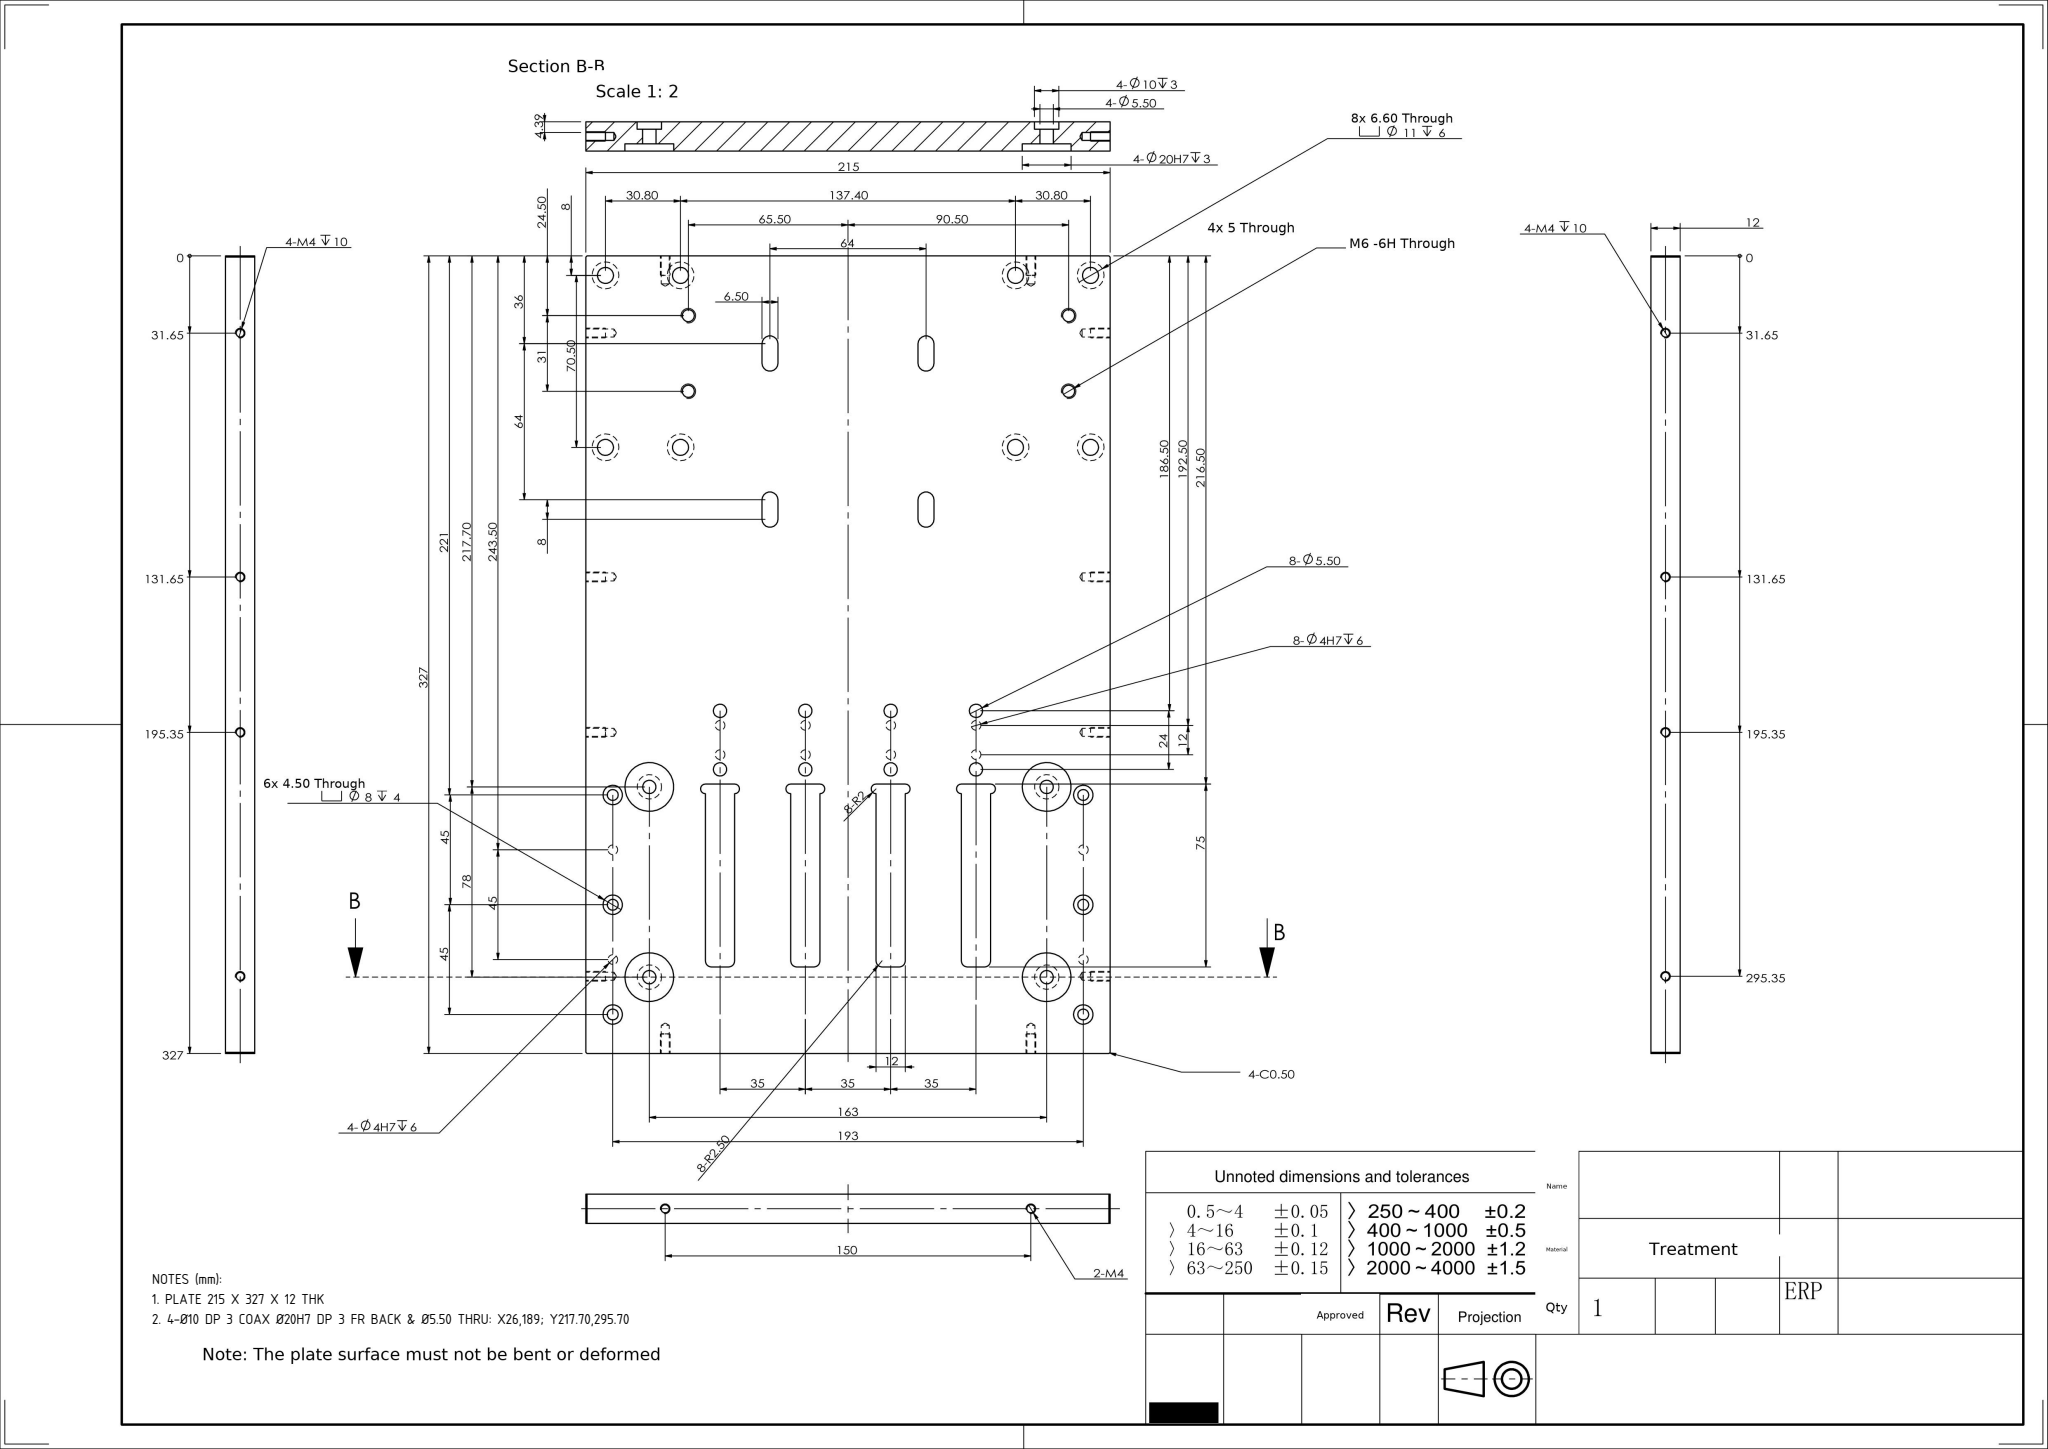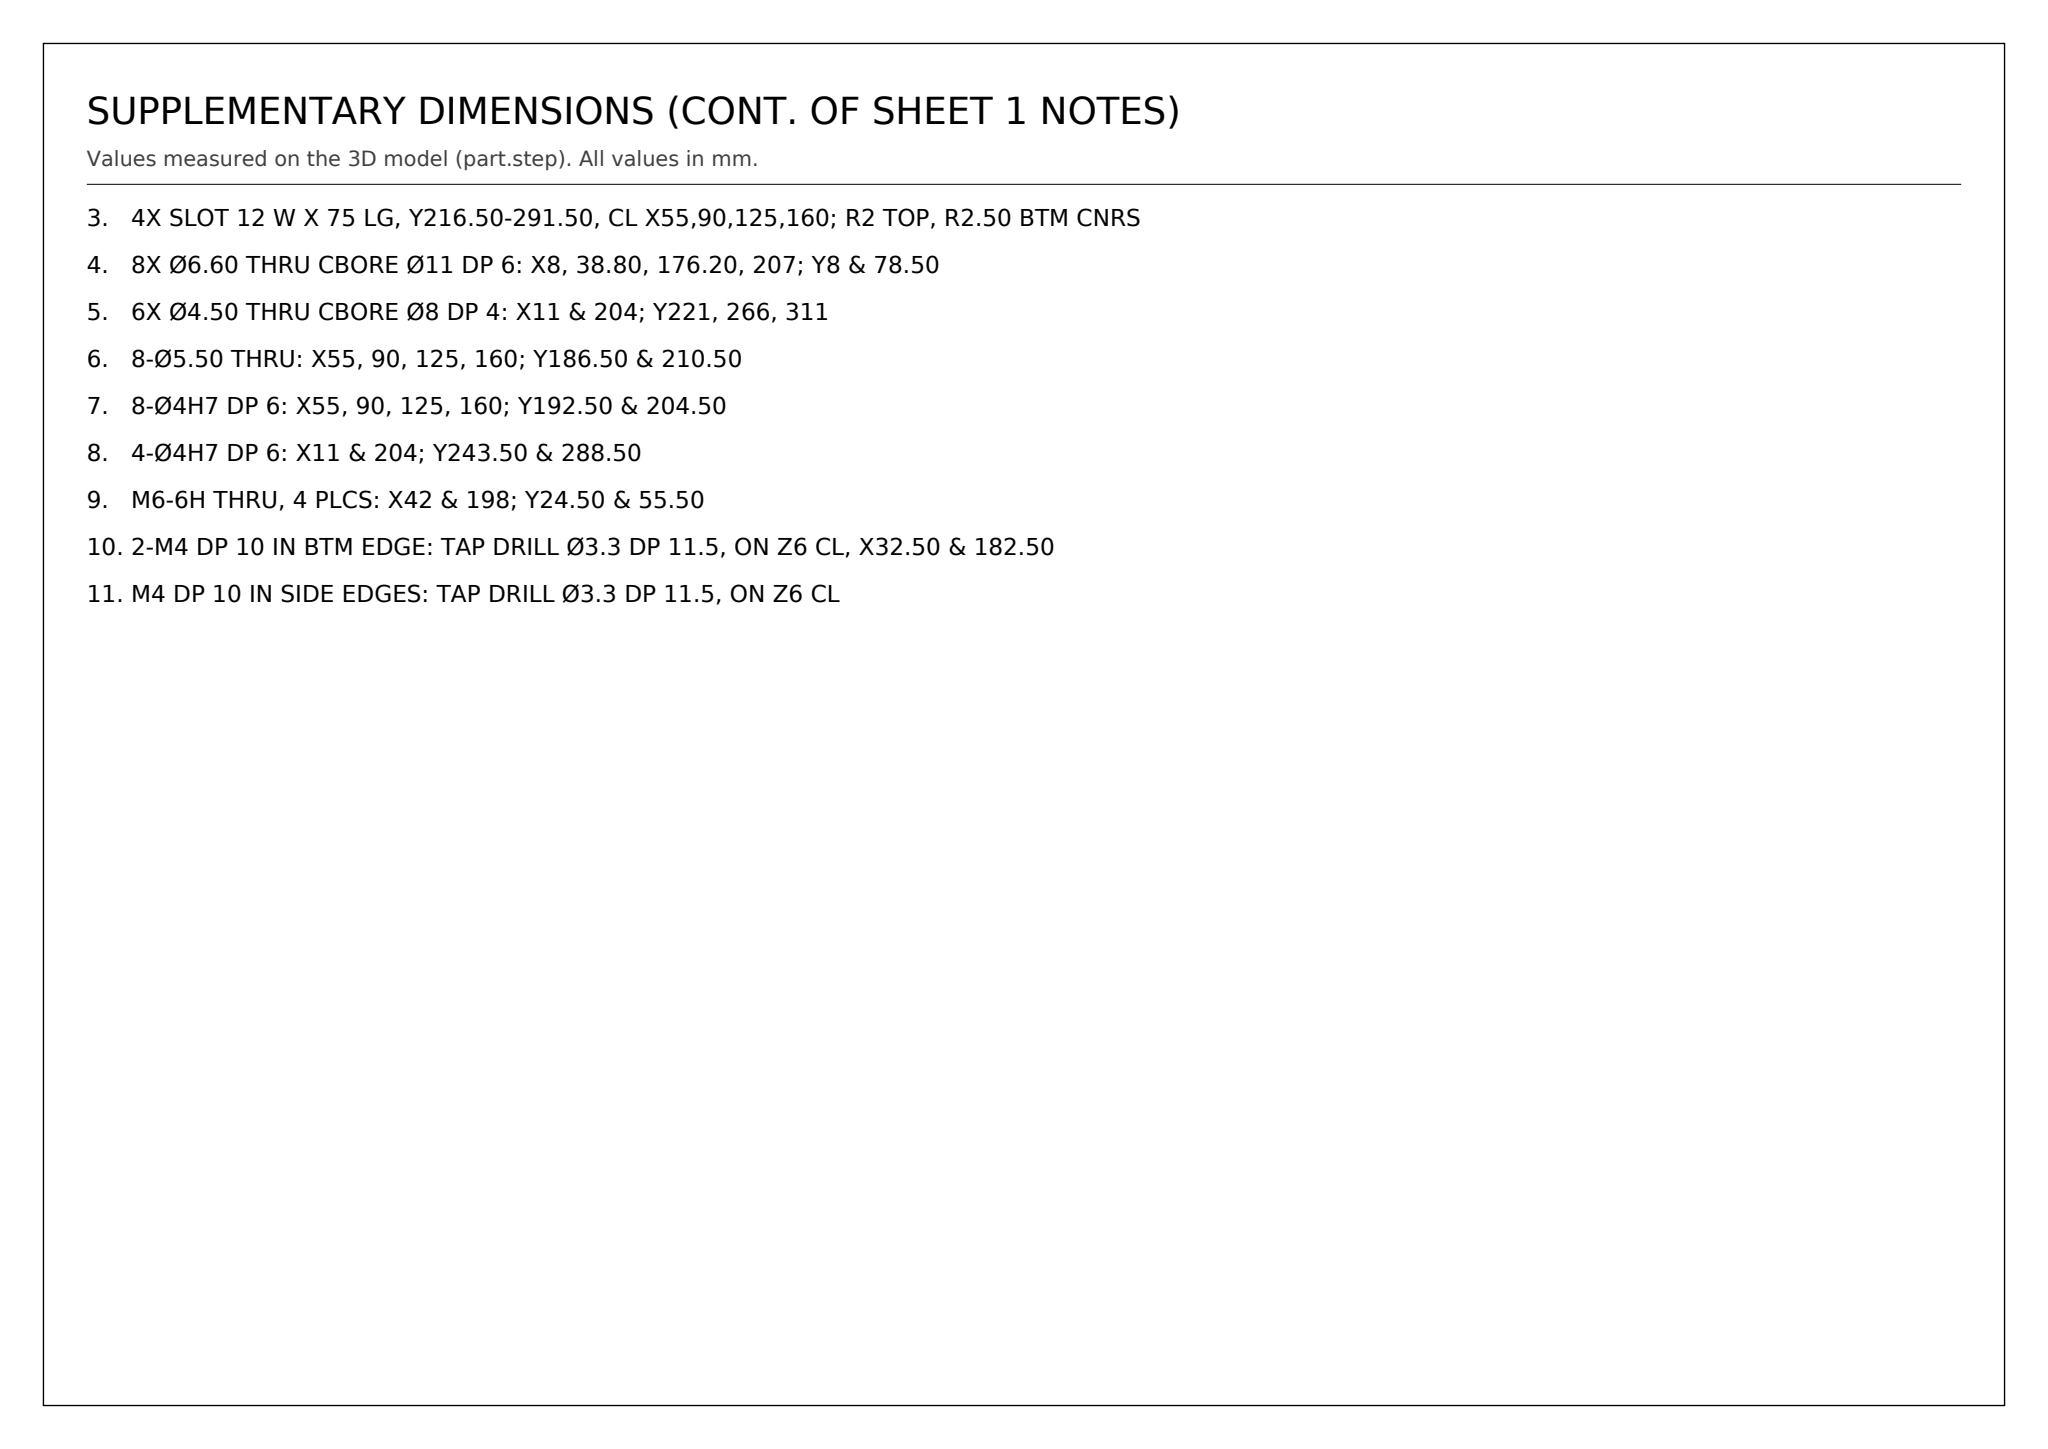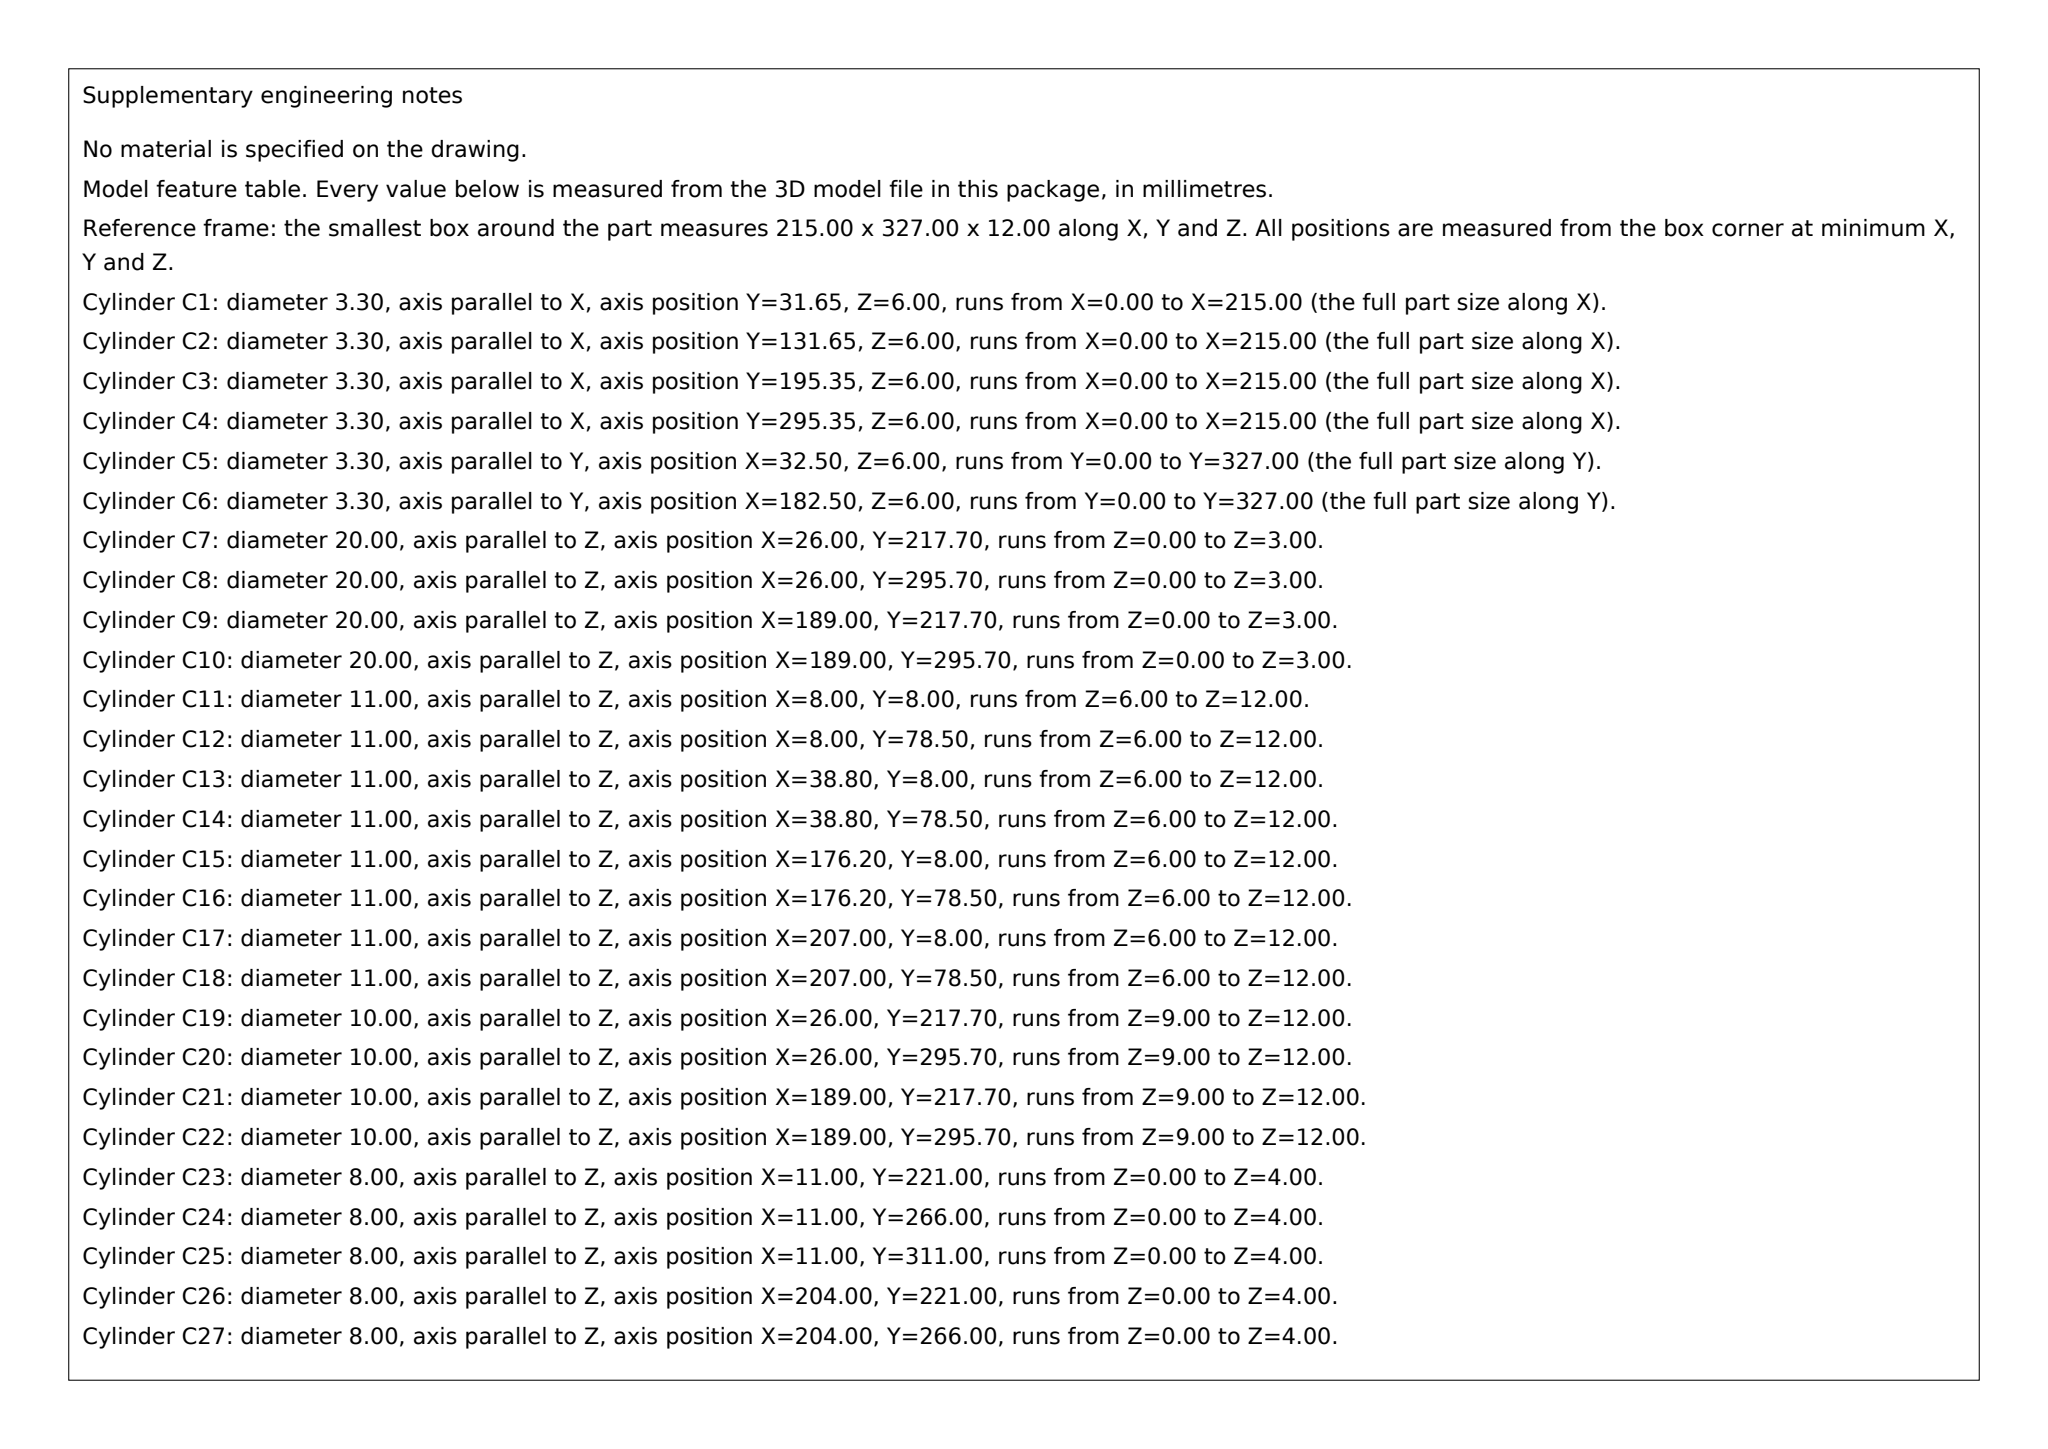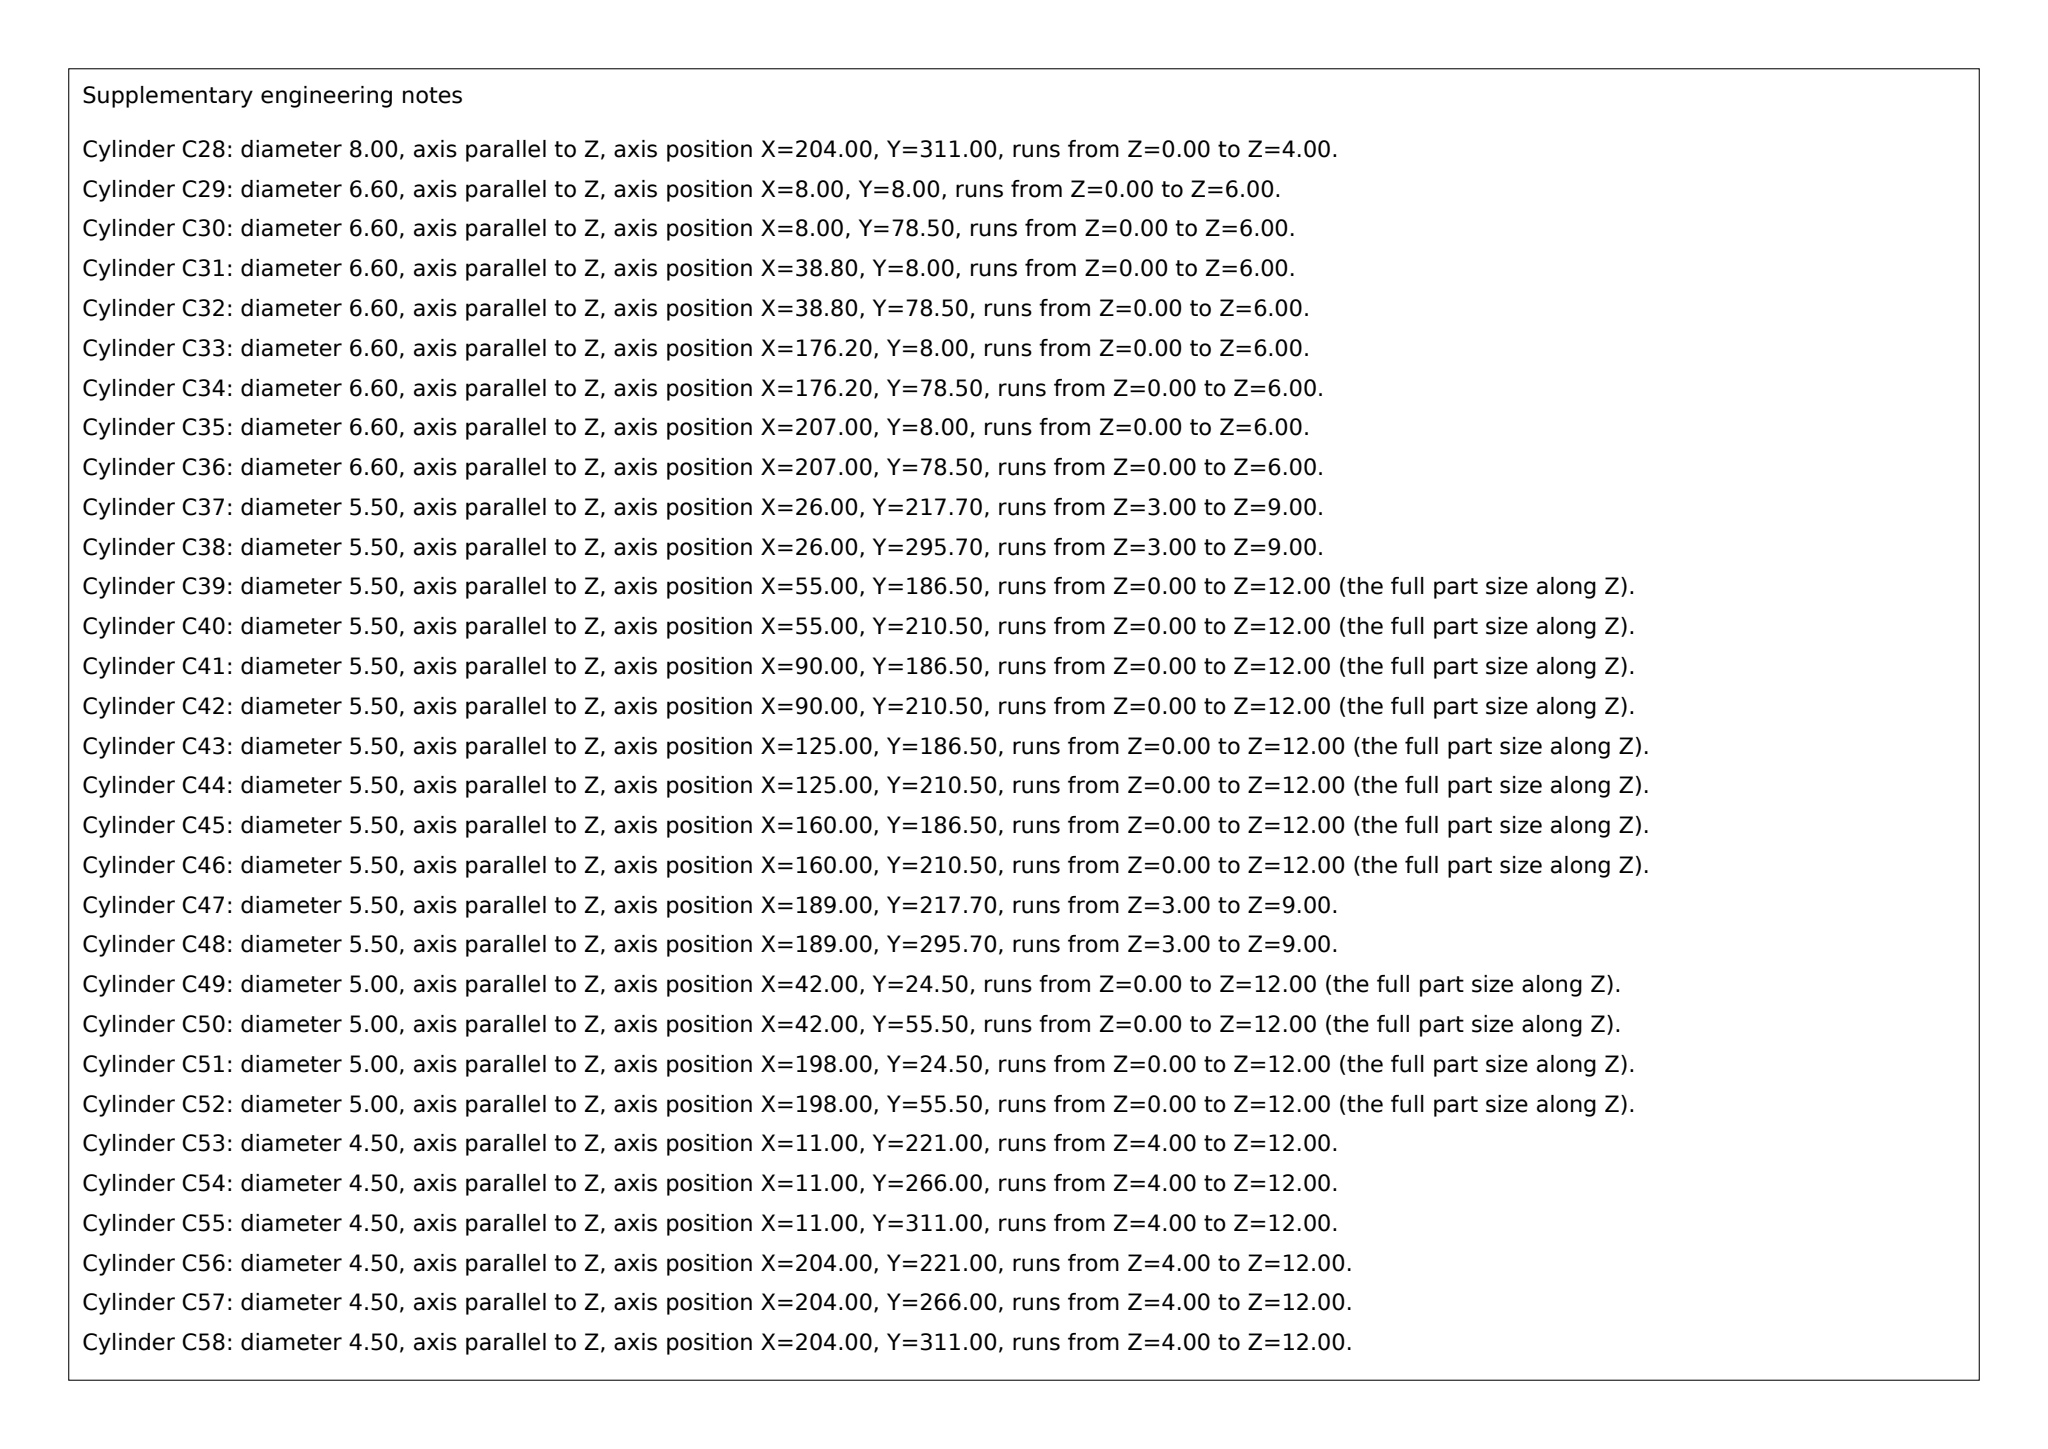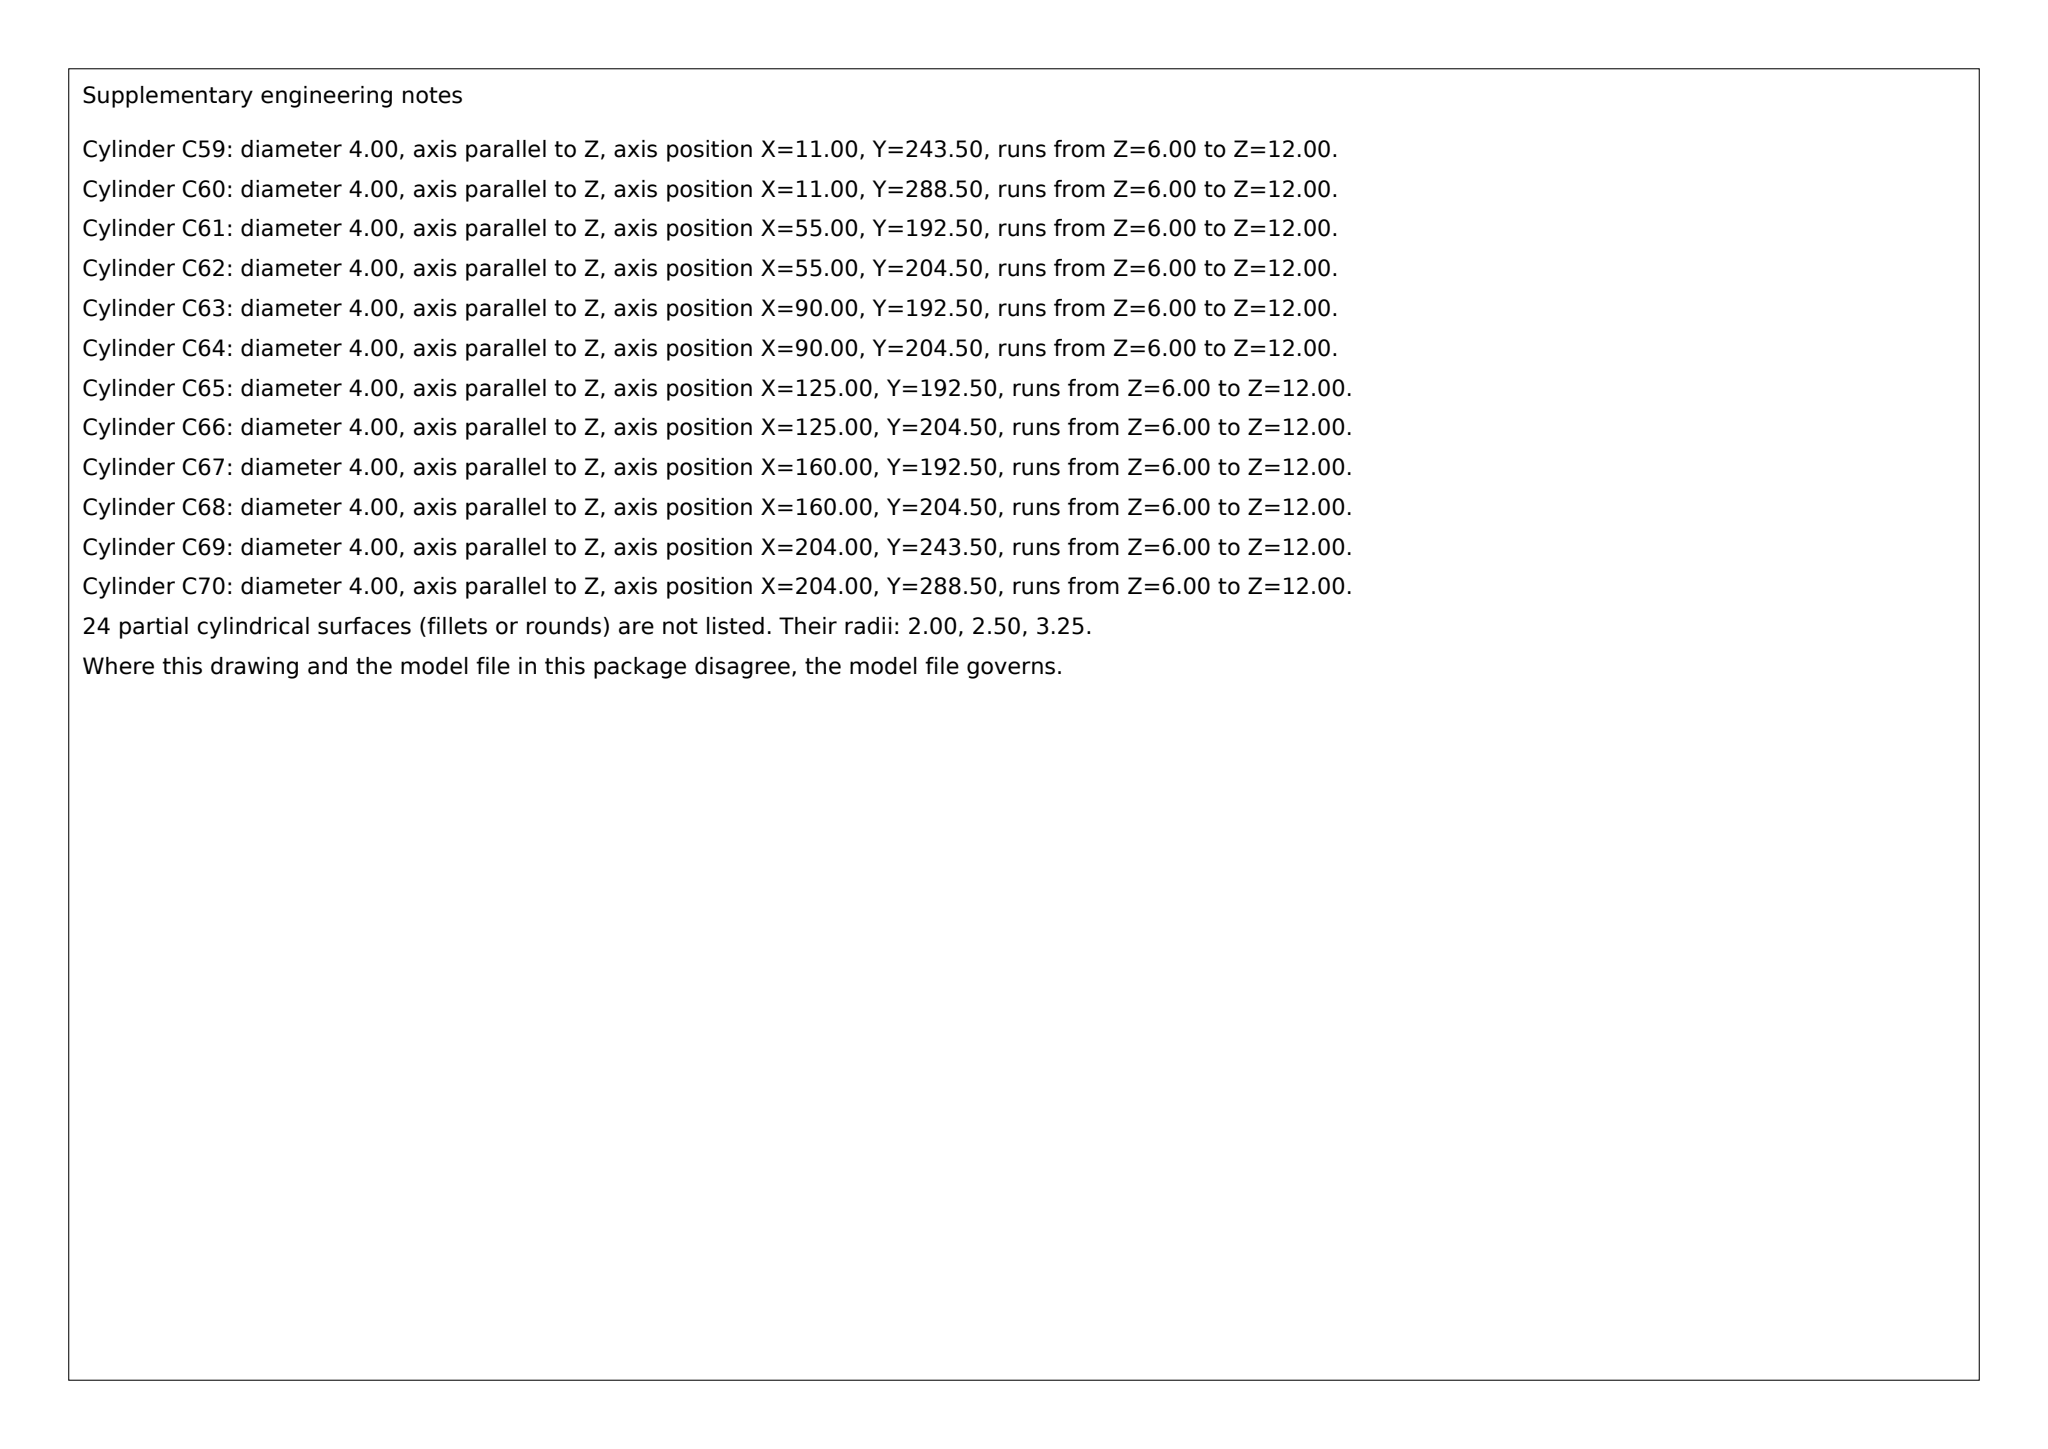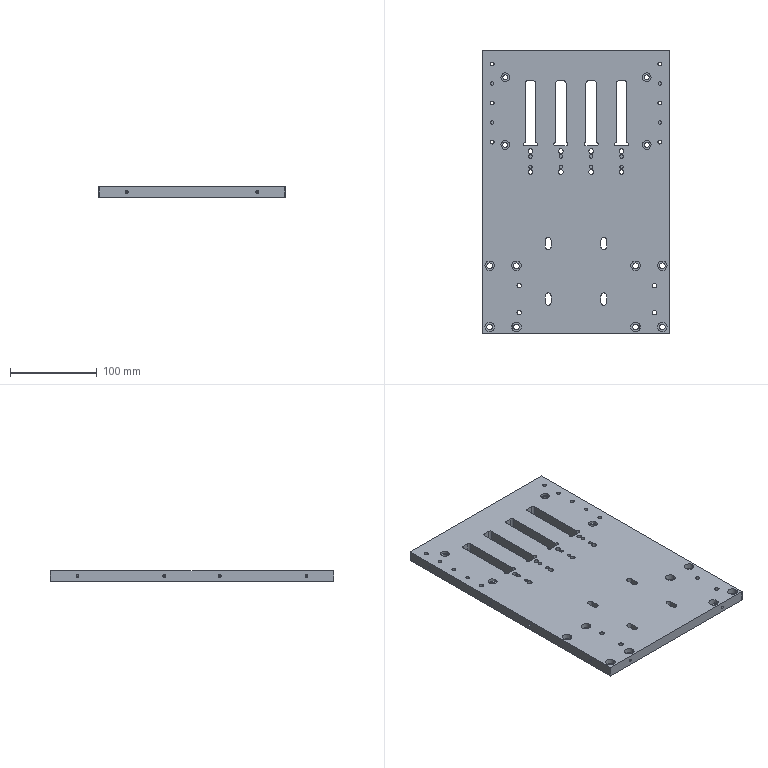Part | SolidWorks | mm | 1 solid | 272 faces | box 215 x 327 x 12 mm | volume 777099 mm3 | cylinder 180 | plane 68 | cone 24 | commonest cylinder face diameters 4 x36 3.3 x24 5.5 x24 11 x16 6.6 x16 5 x16 8 x12 4.5 x12
Drawing notes:
PLATE 215 X 327 X 12 THK | from the solid: bbox_xyz 215 x 327 x 12; z-planes @0 and @12
4-Ø10 DP 3 COAX Ø20H7 DP 3 FR BACK & Ø5.50 THRU: X26,189; Y217.70,295.70 | from the solid: Ø10 L3 at [26,217.7],[26,295.7],[189,217.7],[189,295.7]; z-planes @3 (4x) & @9 (4x); Ø5.5 L6 coax
4X SLOT 12 W X 75 LG, Y216.50-291.50, CL X55,90,125,160; R2 TOP, R2.50 BTM CNRS | from the solid: y-planes 216.5 (4x) & 291.5 (4x); x-planes 49/61, 84/96, 119/131, 154/166; Ø4 L12 cnr radii at y218.5; Ø5 L12 cnr radii at y289
8X Ø6.60 THRU CBORE Ø11 DP 6: X8, 38.80, 176.20, 207; Y8 & 78.50 | from the solid: Ø6.6 L6 at x=8,38.8,176.2,207 with y=8 and 78.5 (8 holes)
6X Ø4.50 THRU CBORE Ø8 DP 4: X11 & 204; Y221, 266, 311 | from the solid: Ø4.5 L8 + Ø8 L4 at [11,221],[11,266],[11,311],[204,221],[204,266],[204,311]
8-Ø5.50 THRU: X55, 90, 125, 160; Y186.50 & 210.50 | from the solid: Ø5.5 L12 at [55,186.5],[55,210.5],[90,...],[125,...],[160,...]
8-Ø4H7 DP 6: X55, 90, 125, 160; Y192.50 & 204.50 | from the solid: Ø4.0 L6 at [55,192.5],[55,204.5],[90,...],[125,...],[160,...]
4-Ø4H7 DP 6: X11 & 204; Y243.50 & 288.50 | from the solid: Ø4.0 L6 at [11,243.5],[11,288.5],[204,243.5],[204,288.5]
M6-6H THRU, 4 PLCS: X42 & 198; Y24.50 & 55.50 | from the solid: Ø5.0 thru (L=12) at [42,24.5],[42,55.5],[198,24.5],[198,55.5] = M6 minor dia
2-M4 DP 10 IN BTM EDGE: TAP DRILL Ø3.3 DP 11.5, ON Z6 CL, X32.50 & 182.50 | from the solid: Ø3.3 cyls axis y at [32.5,-,6.0] & [182.5,-,6.0], L11.5, 118° drill point; 150 spacing = 182.5-32.5
M4 DP 10 IN SIDE EDGES: TAP DRILL Ø3.3 DP 11.5, ON Z6 CL | from the solid: Ø3.3 cyls axis x at y=31.65,131.65,195.35,295.35, z=6.0, L11.5; 118° drill point cone
build123d program:
from build123d import *

# Parameters (mm, degrees)
SKETCH1_W                                       = 215
SKETCH1_H                                       = 327
BOSS_EXTRUDE1_DEPTH                             = 12
M5_HEX_SOCKET_HEAD_CAP_SCREW_CBORE1_D           = 5.5
M5_HEX_SOCKET_HEAD_CAP_SCREW_CBORE1_CBORE_D     = 10
M5_HEX_SOCKET_HEAD_CAP_SCREW_CBORE1_CBORE_DEPTH = 3
SKETCH8_R                                       = 10
CUT_EXTRUDE1_DEPTH                              = 3
SKETCH9_W                                       = 12
SKETCH9_H                                       = 75
CUT_EXTRUDE2_DEPTH                              = 345.426
F_5_5_5_5_DIAMETER_HOLE1_D                      = 5.5
SKETCH24_R                                      = 2
CUT_EXTRUDE10_DEPTH                             = 6
FILLET1_R                                       = 2.5
SKETCH25_R                                      = 2
CUT_EXTRUDE11_DEPTH                             = 345.426
M4_HEX_SOCKET_HEAD_CAP_SCREW_CBORE1_D           = 4.5
M4_HEX_SOCKET_HEAD_CAP_SCREW_CBORE1_CBORE_D     = 8
M4_HEX_SOCKET_HEAD_CAP_SCREW_CBORE1_CBORE_DEPTH = 4
SKETCH28_R                                      = 2
CUT_EXTRUDE12_DEPTH                             = 6
CHAMFER1_SIZE                                   = 0.5
M6_TAPPED_HOLE1_D                               = 5
CUT_EXTRUDE16_DEPTH                             = 345.426
M6_HEX_SOCKET_HEAD_CAP_SCREW_CBORE1_D           = 6.6
M6_HEX_SOCKET_HEAD_CAP_SCREW_CBORE1_CBORE_D     = 11
M6_HEX_SOCKET_HEAD_CAP_SCREW_CBORE1_CBORE_DEPTH = 6
M4_TAPPED_HOLE1_D                               = 3.3
M4_TAPPED_HOLE1_DEPTH                           = 11.5
M4_TAPPED_HOLE1_TIP                             = 0.9914
M4_TAPPED_HOLE2_D                               = 3.3
M4_TAPPED_HOLE2_DEPTH                           = 11.5
M4_TAPPED_HOLE2_TIP                             = 0.9914
M4_TAPPED_HOLE3_D                               = 3.3
M4_TAPPED_HOLE3_DEPTH                           = 11.5
M4_TAPPED_HOLE3_TIP                             = 0.9914
M4_TAPPED_HOLE4_D                               = 3.3
M4_TAPPED_HOLE4_DEPTH                           = 11.5
M4_TAPPED_HOLE4_TIP                             = 0.9914


with BuildPart() as part:
    # Sketch1 → Boss-Extrude1 (new body)
    with BuildSketch(Plane.XY):
        with Locations((0, 163.5)):
            Rectangle(SKETCH1_W, SKETCH1_H)
    extrude(amount=BOSS_EXTRUDE1_DEPTH)

    # M5 Hex Socket Head Cap Screw CBORE1 (through all)
    with Locations(Plane(origin=(-81.5, 295.7, 12), x_dir=(1, 0, 0), z_dir=(0, 0, 1))):
        with Locations((0, 0), (163, 0), (0, -78), (163, -78)):
            CounterBoreHole(M5_HEX_SOCKET_HEAD_CAP_SCREW_CBORE1_D / 2, M5_HEX_SOCKET_HEAD_CAP_SCREW_CBORE1_CBORE_D / 2, M5_HEX_SOCKET_HEAD_CAP_SCREW_CBORE1_CBORE_DEPTH)

    # Sketch8 → Cut-Extrude1 (cut)
    with BuildSketch(Plane(origin=(0, 0, 0), x_dir=(-1, 0, 0), z_dir=(0, 0, -1))):
        with Locations((-81.5, 295.7)):
            Circle(SKETCH8_R)
        with Locations((81.5, 295.7)):
            Circle(SKETCH8_R)
        with Locations((-81.5, 217.7)):
            Circle(SKETCH8_R)
        with Locations((81.5, 217.7)):
            Circle(SKETCH8_R)
    extrude(amount=-CUT_EXTRUDE1_DEPTH, mode=Mode.SUBTRACT)

    # Sketch9 → Cut-Extrude2 (cut, through all)
    with BuildSketch(Plane.XY.offset(12)):
        with Locations((-52.5, 254)):
            Rectangle(SKETCH9_W, SKETCH9_H)
        with Locations((-17.5, 254)):
            Rectangle(SKETCH9_W, SKETCH9_H)
        with Locations((17.5, 254)):
            Rectangle(SKETCH9_W, SKETCH9_H)
        with Locations((52.5, 254)):
            Rectangle(SKETCH9_W, SKETCH9_H)
    extrude(amount=-CUT_EXTRUDE2_DEPTH, mode=Mode.SUBTRACT)

    # 5.5 _5.5_ Diameter Hole1 (through all)
    with Locations(Plane(origin=(17.5, 210.5, 0), x_dir=(-1, 0, 0), z_dir=(0, 0, -1))):
        with Locations((0, 0), (0, -24), (35, 0), (35, -24), (70, 0), (70, -24), (-35, 0), (-35, -24)):
            Hole(F_5_5_5_5_DIAMETER_HOLE1_D / 2)

    # Sketch24 → Cut-Extrude10 (cut)
    with BuildSketch(Plane.XY.offset(12)):
        with Locations((52.5, 204.5)):
            Circle(SKETCH24_R)
        with Locations((52.5, 192.5)):
            Circle(SKETCH24_R)
        with Locations((17.5, 204.5)):
            Circle(SKETCH24_R)
        with Locations((17.5, 192.5)):
            Circle(SKETCH24_R)
        with Locations((-17.5, 204.5)):
            Circle(SKETCH24_R)
        with Locations((-17.5, 192.5)):
            Circle(SKETCH24_R)
        with Locations((-52.5, 204.5)):
            Circle(SKETCH24_R)
        with Locations((-52.5, 192.5)):
            Circle(SKETCH24_R)
    extrude(amount=-CUT_EXTRUDE10_DEPTH, mode=Mode.SUBTRACT)

    # Fillet1
    fillet1_edges = [part.edges().sort_by_distance(p)[0] for p in [
        (46.5, 291.5, 6),
        (58.5, 291.5, 6),
        (-58.5, 291.5, 6),
        (-46.5, 291.5, 6),
        (-23.5, 291.5, 6),
        (-11.5, 291.5, 6),
        (11.5, 291.5, 6),
        (23.5, 291.5, 6),
    ]]
    fillet(fillet1_edges, radius=FILLET1_R)

    # Sketch25 → Cut-Extrude11 (cut, through all)
    with BuildSketch(Plane.XY.offset(12)):
        with Locations((23.5, 218.5)):
            Circle(SKETCH25_R)
        with Locations((11.5, 218.5)):
            Circle(SKETCH25_R)
        with Locations((-11.5, 218.5)):
            Circle(SKETCH25_R)
        with Locations((-23.5, 218.5)):
            Circle(SKETCH25_R)
        with Locations((-46.5, 218.5)):
            Circle(SKETCH25_R)
        with Locations((-58.5, 218.5)):
            Circle(SKETCH25_R)
        with Locations((46.5, 218.5)):
            Circle(SKETCH25_R)
        with Locations((58.5, 218.5)):
            Circle(SKETCH25_R)
    extrude(amount=-CUT_EXTRUDE11_DEPTH, mode=Mode.SUBTRACT)

    # M4 Hex Socket Head Cap Screw CBORE1 (through all)
    with Locations(Plane(origin=(0, 0, 0), x_dir=(-1, 0, 0), z_dir=(0, 0, -1))):
        with Locations((96.5, 311), (96.5, 266), (96.5, 221), (-96.5, 311), (-96.5, 266), (-96.5, 221)):
            CounterBoreHole(M4_HEX_SOCKET_HEAD_CAP_SCREW_CBORE1_D / 2, M4_HEX_SOCKET_HEAD_CAP_SCREW_CBORE1_CBORE_D / 2, M4_HEX_SOCKET_HEAD_CAP_SCREW_CBORE1_CBORE_DEPTH)

    # Sketch28 → Cut-Extrude12 (cut)
    with BuildSketch(Plane.XY.offset(12)):
        with Locations((-96.5, 288.5)):
            Circle(SKETCH28_R)
        with Locations((-96.5, 243.5)):
            Circle(SKETCH28_R)
        with Locations((96.5, 288.5)):
            Circle(SKETCH28_R)
        with Locations((96.5, 243.5)):
            Circle(SKETCH28_R)
    extrude(amount=-CUT_EXTRUDE12_DEPTH, mode=Mode.SUBTRACT)

    # Chamfer1
    chamfer1_edges = [part.edges().sort_by_distance(p)[0] for p in [
        (-107.5, 327, 6),
        (107.5, 327, 6),
        (107.5, 0, 6),
        (-107.5, 0, 6),
    ]]
    chamfer(chamfer1_edges, length=CHAMFER1_SIZE)

    # M6 Tapped Hole1 (through all)
    with Locations(Plane(origin=(-65.5, 24.5, 12), x_dir=(1, 0, 0), z_dir=(0, 0, 1))):
        with Locations((0, 0), (0, 31), (156, 0), (156, 31)):
            Hole(M6_TAPPED_HOLE1_D / 2)

    # Sketch38 → Cut-Extrude16 (cut, through all)
    with BuildSketch(Plane.XY.offset(12)):
        with BuildLine():
            Line((-28.75, 108), (-28.75, 100))
            ThreePointArc((-28.75, 100), (-32, 96.75), (-35.25, 100))
            Line((-35.25, 100), (-35.25, 108))
            ThreePointArc((-35.25, 108), (-32, 111.25), (-28.75, 108))
        make_face()
        with BuildLine():
            Line((35.25, 108), (35.25, 100))
            ThreePointArc((35.25, 100), (32, 96.75), (28.75, 100))
            Line((28.75, 100), (28.75, 108))
            ThreePointArc((28.75, 108), (32, 111.25), (35.25, 108))
        make_face()
        with BuildLine():
            Line((35.25, 44), (35.25, 36))
            ThreePointArc((35.25, 36), (32, 32.75), (28.75, 36))
            Line((28.75, 36), (28.75, 44))
            ThreePointArc((28.75, 44), (32, 47.25), (35.25, 44))
        make_face()
        with BuildLine():
            Line((-28.75, 44), (-28.75, 36))
            ThreePointArc((-28.75, 36), (-32, 32.75), (-35.25, 36))
            Line((-35.25, 36), (-35.25, 44))
            ThreePointArc((-35.25, 44), (-32, 47.25), (-28.75, 44))
        make_face()
    extrude(amount=-CUT_EXTRUDE16_DEPTH, mode=Mode.SUBTRACT)

    # M6 Hex Socket Head Cap Screw CBORE1 (through all)
    with Locations(Plane(origin=(-99.5, 8, 12), x_dir=(1, 0, 0), z_dir=(0, 0, 1))):
        with Locations((0, 0), (30.8, 0), (0, 70.5), (30.8, 70.5), (168.2, 0), (199, 0), (168.2, 70.5), (199, 70.5)):
            CounterBoreHole(M6_HEX_SOCKET_HEAD_CAP_SCREW_CBORE1_D / 2, M6_HEX_SOCKET_HEAD_CAP_SCREW_CBORE1_CBORE_D / 2, M6_HEX_SOCKET_HEAD_CAP_SCREW_CBORE1_CBORE_DEPTH)

    # M4 Tapped Hole1
    with Locations(Plane(origin=(0, 0, 0), x_dir=(-1, 0, 0), z_dir=(0, -1, 0))):
        with Locations((75, -6), (-75, -6)):
            Hole(M4_TAPPED_HOLE1_D / 2, depth=M4_TAPPED_HOLE1_DEPTH)
            with Locations((0, 0, -(M4_TAPPED_HOLE1_DEPTH + M4_TAPPED_HOLE1_TIP / 2))):  # 118° drill point
                Cone(0, M4_TAPPED_HOLE1_D / 2, M4_TAPPED_HOLE1_TIP, mode=Mode.SUBTRACT)

    # M4 Tapped Hole2
    with Locations(Plane(origin=(107.5, 0, 0), x_dir=(0, 0, -1), z_dir=(1, 0, 0))):
        with Locations((-6, 31.65), (-6, 131.65), (-6, 195.35), (-6, 295.35)):
            Hole(M4_TAPPED_HOLE2_D / 2, depth=M4_TAPPED_HOLE2_DEPTH)
            with Locations((0, 0, -(M4_TAPPED_HOLE2_DEPTH + M4_TAPPED_HOLE2_TIP / 2))):  # 118° drill point
                Cone(0, M4_TAPPED_HOLE2_D / 2, M4_TAPPED_HOLE2_TIP, mode=Mode.SUBTRACT)

    # M4 Tapped Hole3
    with Locations(Plane.ZY.offset(107.5)):
        with Locations((6, 31.65), (6, 131.65), (6, 195.35), (6, 295.35)):
            Hole(M4_TAPPED_HOLE3_D / 2, depth=M4_TAPPED_HOLE3_DEPTH)
            with Locations((0, 0, -(M4_TAPPED_HOLE3_DEPTH + M4_TAPPED_HOLE3_TIP / 2))):  # 118° drill point
                Cone(0, M4_TAPPED_HOLE3_D / 2, M4_TAPPED_HOLE3_TIP, mode=Mode.SUBTRACT)

    # M4 Tapped Hole4
    with Locations(Plane(origin=(0, 327, 0), x_dir=(1, 0, 0), z_dir=(0, 1, 0))):
        with Locations((75, -6), (-75, -6)):
            Hole(M4_TAPPED_HOLE4_D / 2, depth=M4_TAPPED_HOLE4_DEPTH)
            with Locations((0, 0, -(M4_TAPPED_HOLE4_DEPTH + M4_TAPPED_HOLE4_TIP / 2))):  # 118° drill point
                Cone(0, M4_TAPPED_HOLE4_D / 2, M4_TAPPED_HOLE4_TIP, mode=Mode.SUBTRACT)


solid = part.part